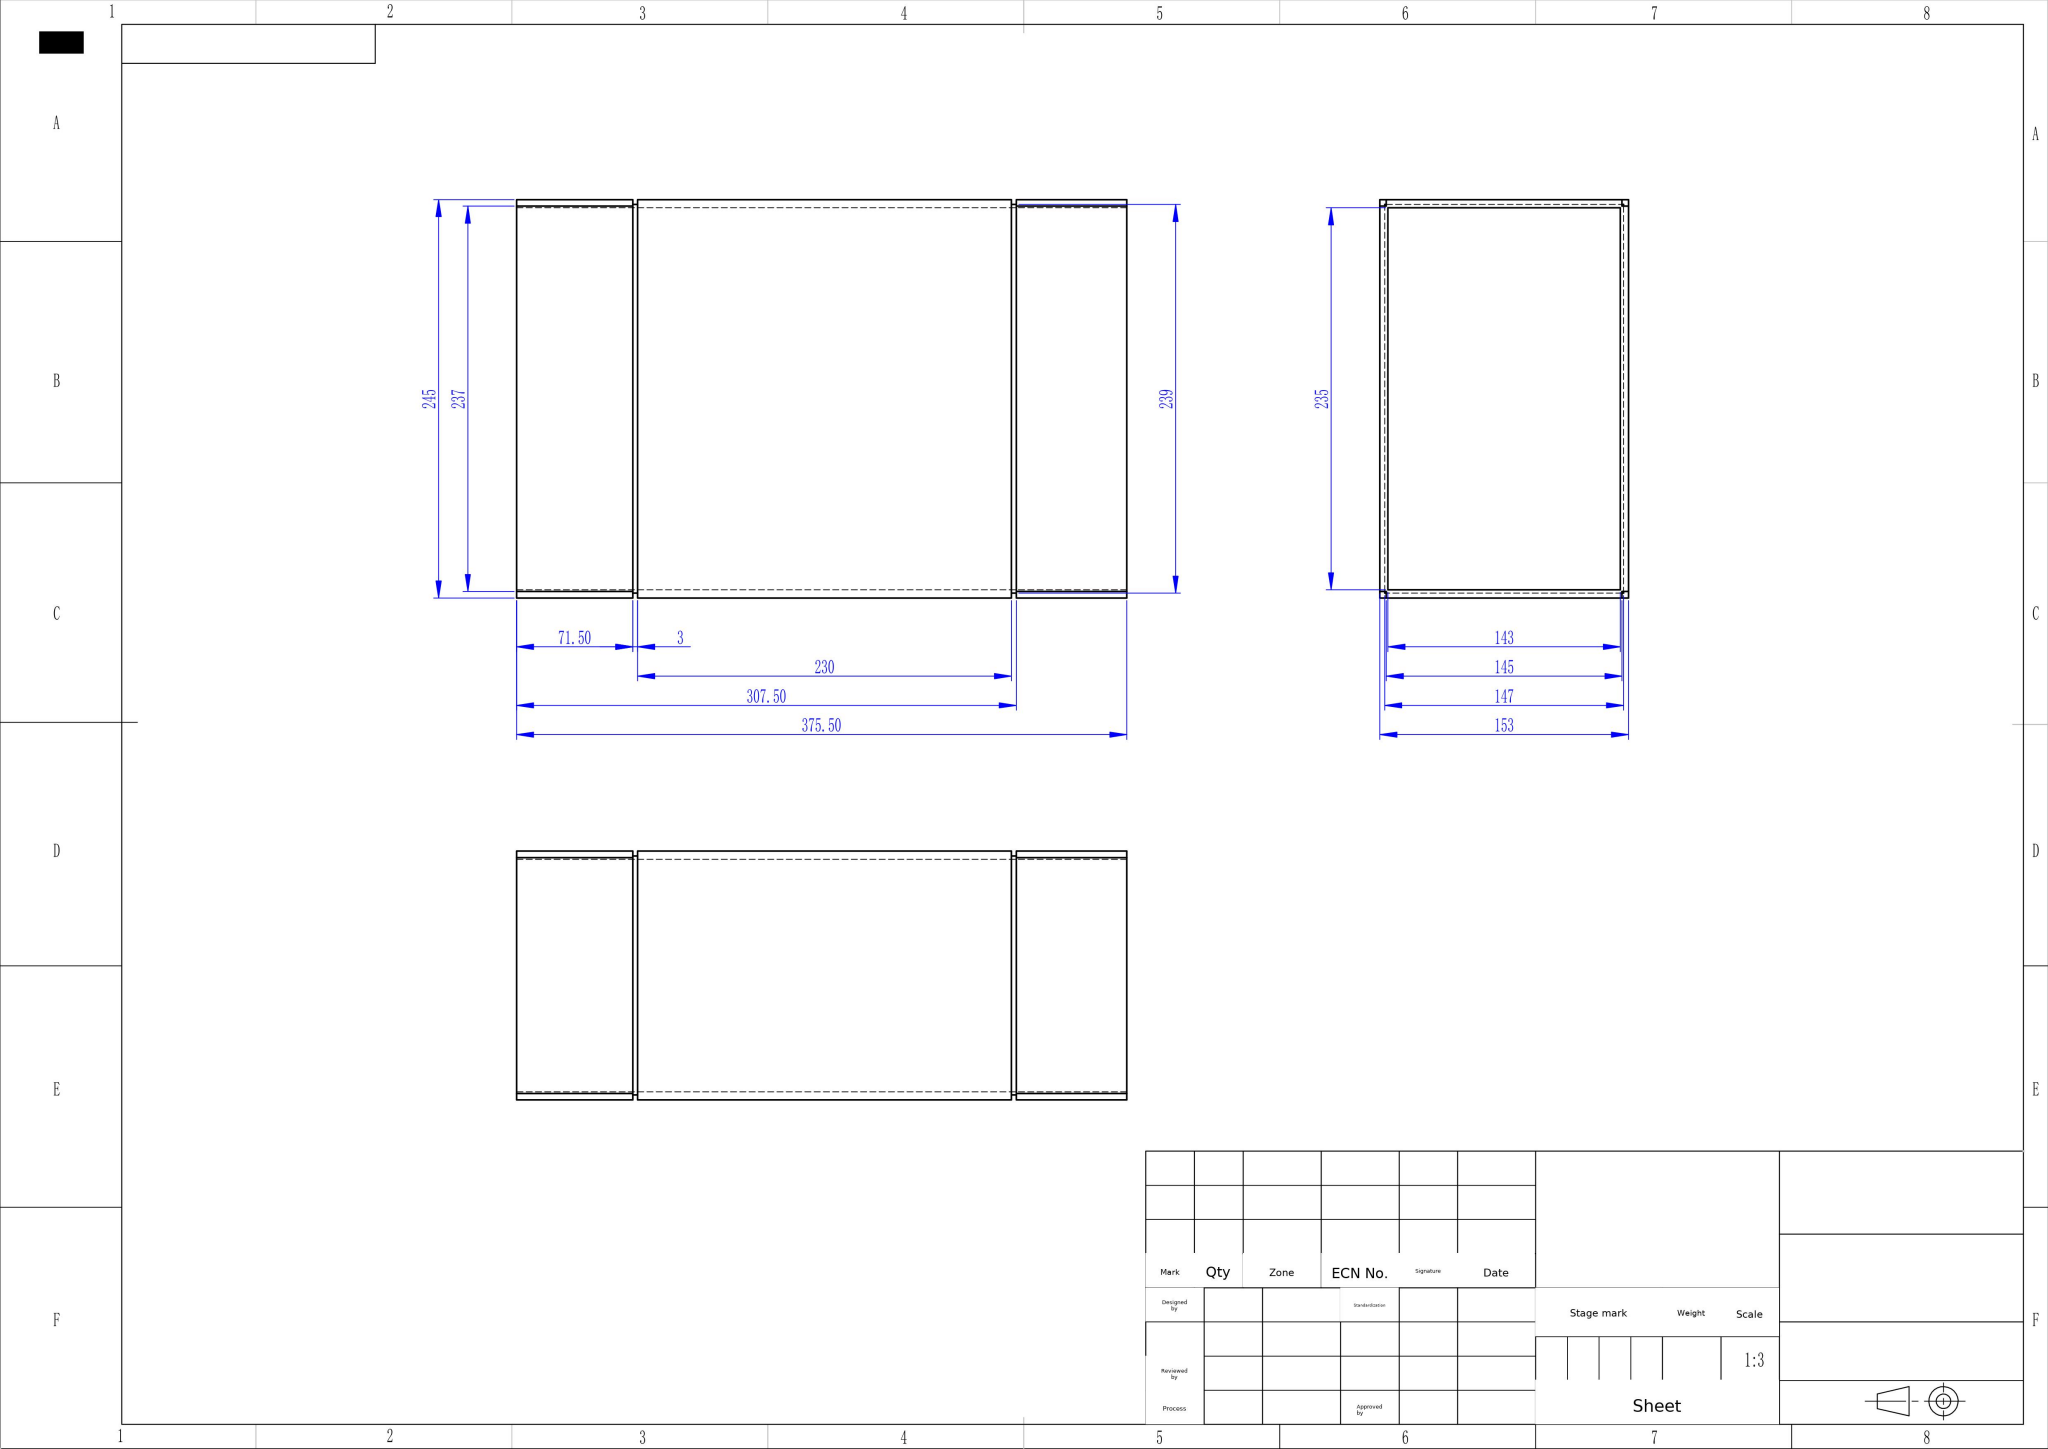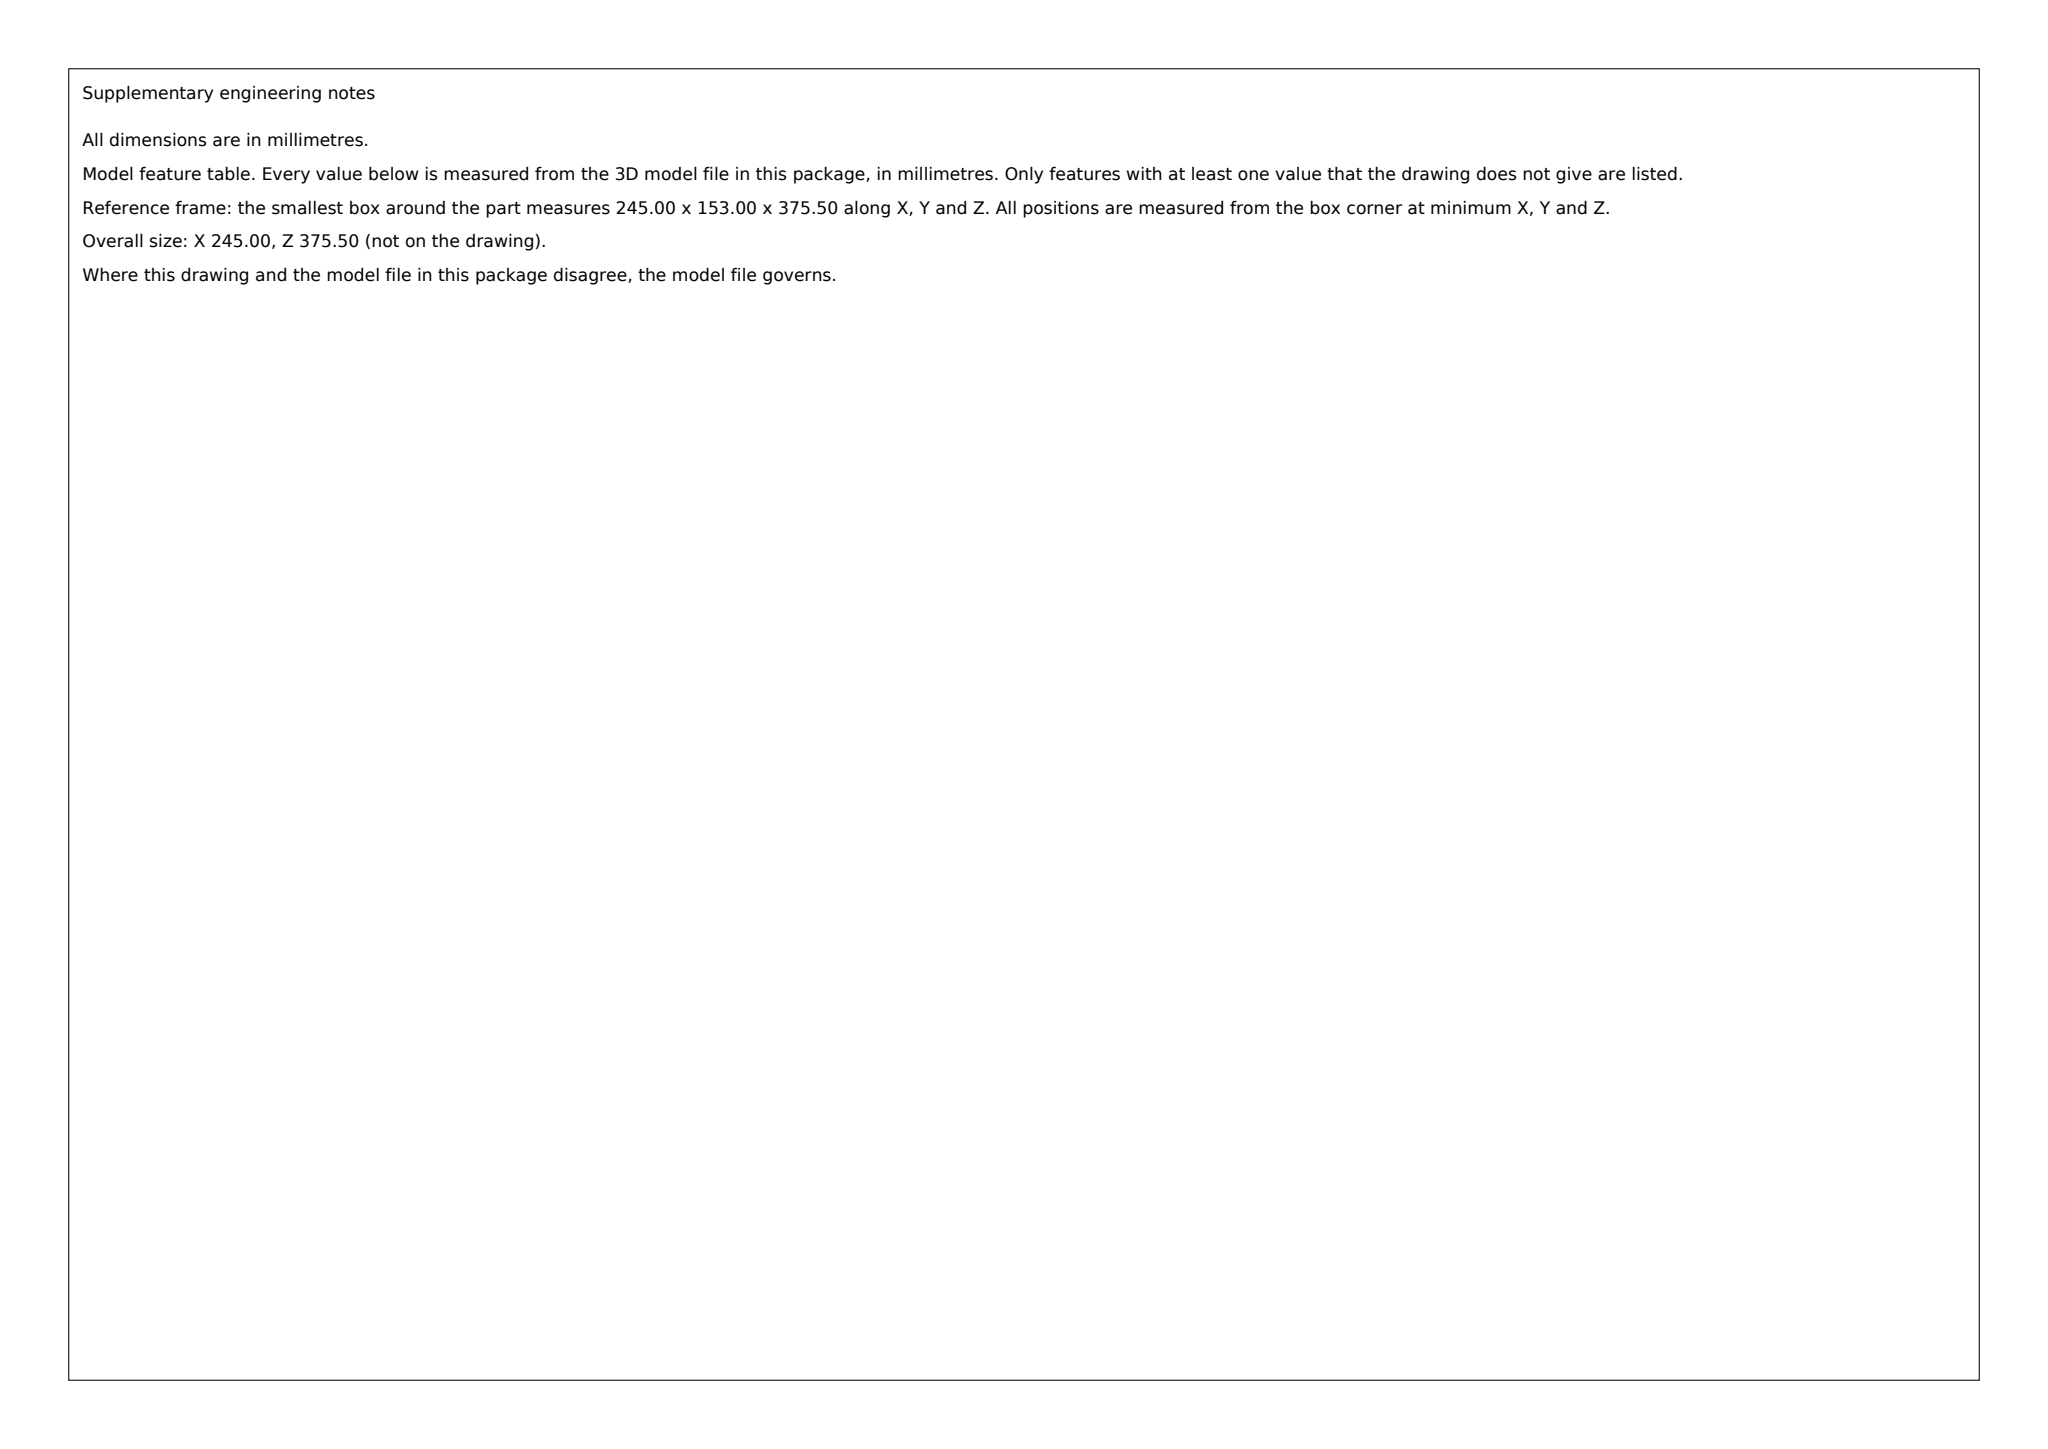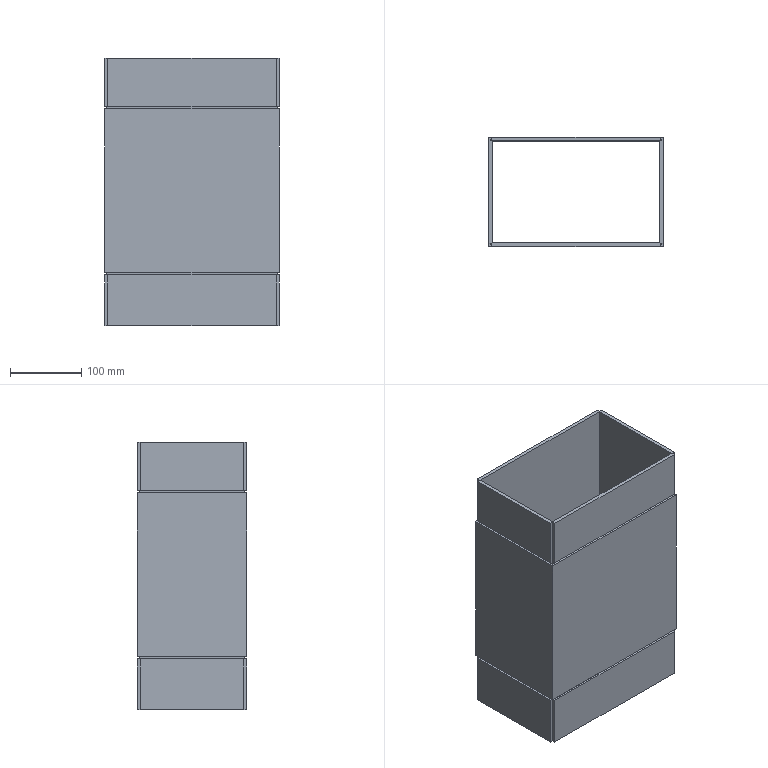Part | SolidWorks | mm | 1 solid | 60 faces | box 245 x 153 x 375.5 mm | volume 1433900 mm3 | plane 60
build123d program:
from build123d import *

# Parameters (mm, degrees)
SKETCH1_W           = 245
SKETCH1_H           = 153
SKETCH1_W_2         = 235
SKETCH1_H_2         = 143
BOSS_EXTRUDE1_DEPTH = 152.25
SKETCH2_W           = 245
SKETCH2_H           = 3
CUT_EXTRUDE1_DEPTH  = 3
SKETCH3_W           = 3
SKETCH3_H           = 150
CUT_EXTRUDE2_DEPTH  = 3
SKETCH4_W           = 242
SKETCH4_H           = 3
CUT_EXTRUDE3_DEPTH  = 3
SKETCH5_W           = 3
SKETCH5_H           = 147
CUT_EXTRUDE4_DEPTH  = 3
SKETCH6_W           = 4
SKETCH6_H           = 4
CUT_EXTRUDE5_DEPTH  = 71.5
SKETCH8_W           = 245
SKETCH8_H           = 153
SKETCH8_W_2         = 235
SKETCH8_H_2         = 143
BOSS_EXTRUDE2_DEPTH = 71


with BuildPart() as part:
    # Sketch1 → Boss-Extrude1 (new, symmetric)
    with BuildSketch(Plane.XY):
        Rectangle(SKETCH1_W, SKETCH1_H)
        Rectangle(SKETCH1_W_2, SKETCH1_H_2, mode=Mode.SUBTRACT)
    extrude(amount=BOSS_EXTRUDE1_DEPTH, both=True)

    # Sketch2 → Cut-Extrude1 (cut)
    with BuildSketch(Plane(origin=(0, 76.5, 0), x_dir=(-1, 0, 0), z_dir=(0, 1, 0))):
        with Locations((0, -79.25)):
            Rectangle(SKETCH2_W, SKETCH2_H)
    cut_extrude1 = extrude(amount=-CUT_EXTRUDE1_DEPTH, mode=Mode.SUBTRACT)

    # Sketch3 → Cut-Extrude2 (cut)
    with BuildSketch(Plane.ZY.offset(122.5)):
        with Locations((-79.25, -1.5)):
            Rectangle(SKETCH3_W, SKETCH3_H)
    cut_extrude2 = extrude(amount=-CUT_EXTRUDE2_DEPTH, mode=Mode.SUBTRACT)

    # Sketch4 → Cut-Extrude3 (cut)
    with BuildSketch(Plane.XZ.offset(76.5)):
        with Locations((1.5, -79.25)):
            Rectangle(SKETCH4_W, SKETCH4_H)
    cut_extrude3 = extrude(amount=-CUT_EXTRUDE3_DEPTH, mode=Mode.SUBTRACT)

    # Sketch5 → Cut-Extrude4 (cut)
    with BuildSketch(Plane(origin=(122.5, 0, 0), x_dir=(0, 0, -1), z_dir=(1, 0, 0))):
        with Locations((79.25, 0)):
            Rectangle(SKETCH5_W, SKETCH5_H)
    cut_extrude4 = extrude(amount=-CUT_EXTRUDE4_DEPTH, mode=Mode.SUBTRACT)

    # Sketch6 → Cut-Extrude5 (cut)
    with BuildSketch(Plane(origin=(0, 0, -152.25), x_dir=(-1, 0, 0), z_dir=(0, 0, -1))):
        with Locations((120.5, 74.5)):
            Rectangle(SKETCH6_W, SKETCH6_H)
        with Locations((120.5, -74.5)):
            Rectangle(SKETCH6_W, SKETCH6_H)
        with Locations((-120.5, -74.5)):
            Rectangle(SKETCH6_W, SKETCH6_H)
        with Locations((-120.5, 74.5)):
            Rectangle(SKETCH6_W, SKETCH6_H)
    cut_extrude5 = extrude(amount=-CUT_EXTRUDE5_DEPTH, mode=Mode.SUBTRACT)

    # Sketch8 → Boss-Extrude2 (add)
    with BuildSketch(Plane.XY.offset(152.25)):
        Rectangle(SKETCH8_W, SKETCH8_H)
        Rectangle(SKETCH8_W_2, SKETCH8_H_2, mode=Mode.SUBTRACT)
    extrude(amount=BOSS_EXTRUDE2_DEPTH)

    # Mirror2: Cut-Extrude1, Cut-Extrude2, Cut-Extrude3, Cut-Extrude4, Cut-Extrude5 across plane
    add(cut_extrude1.mirror(Plane.XY.offset(37.25)), mode=Mode.SUBTRACT)
    add(cut_extrude2.mirror(Plane.XY.offset(37.25)), mode=Mode.SUBTRACT)
    add(cut_extrude3.mirror(Plane.XY.offset(37.25)), mode=Mode.SUBTRACT)
    add(cut_extrude4.mirror(Plane.XY.offset(37.25)), mode=Mode.SUBTRACT)
    add(cut_extrude5.mirror(Plane.XY.offset(37.25)), mode=Mode.SUBTRACT)


solid = part.part